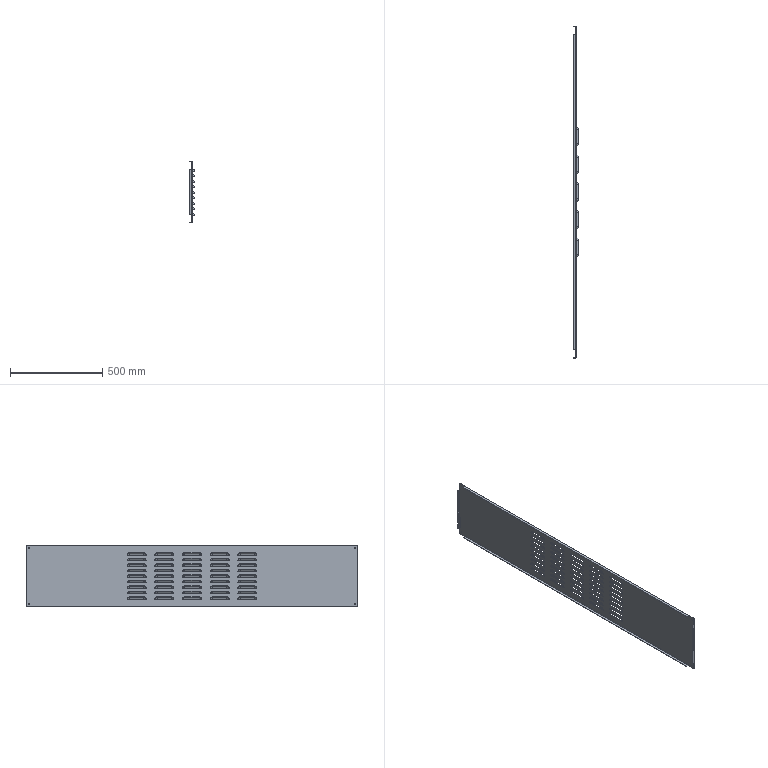Component | SolidWorks | AX00-100.1.1-1_19.1.1-1 | 1 solid | 573 faces | volume 1353721 mm3 | sphere 180 | plane 152 | cylinder 151 | torus 90 | commonest cylinder face diameters 24 x45 4 x45 28 x45 4.5 x8 5.473 x4 1.473 x4